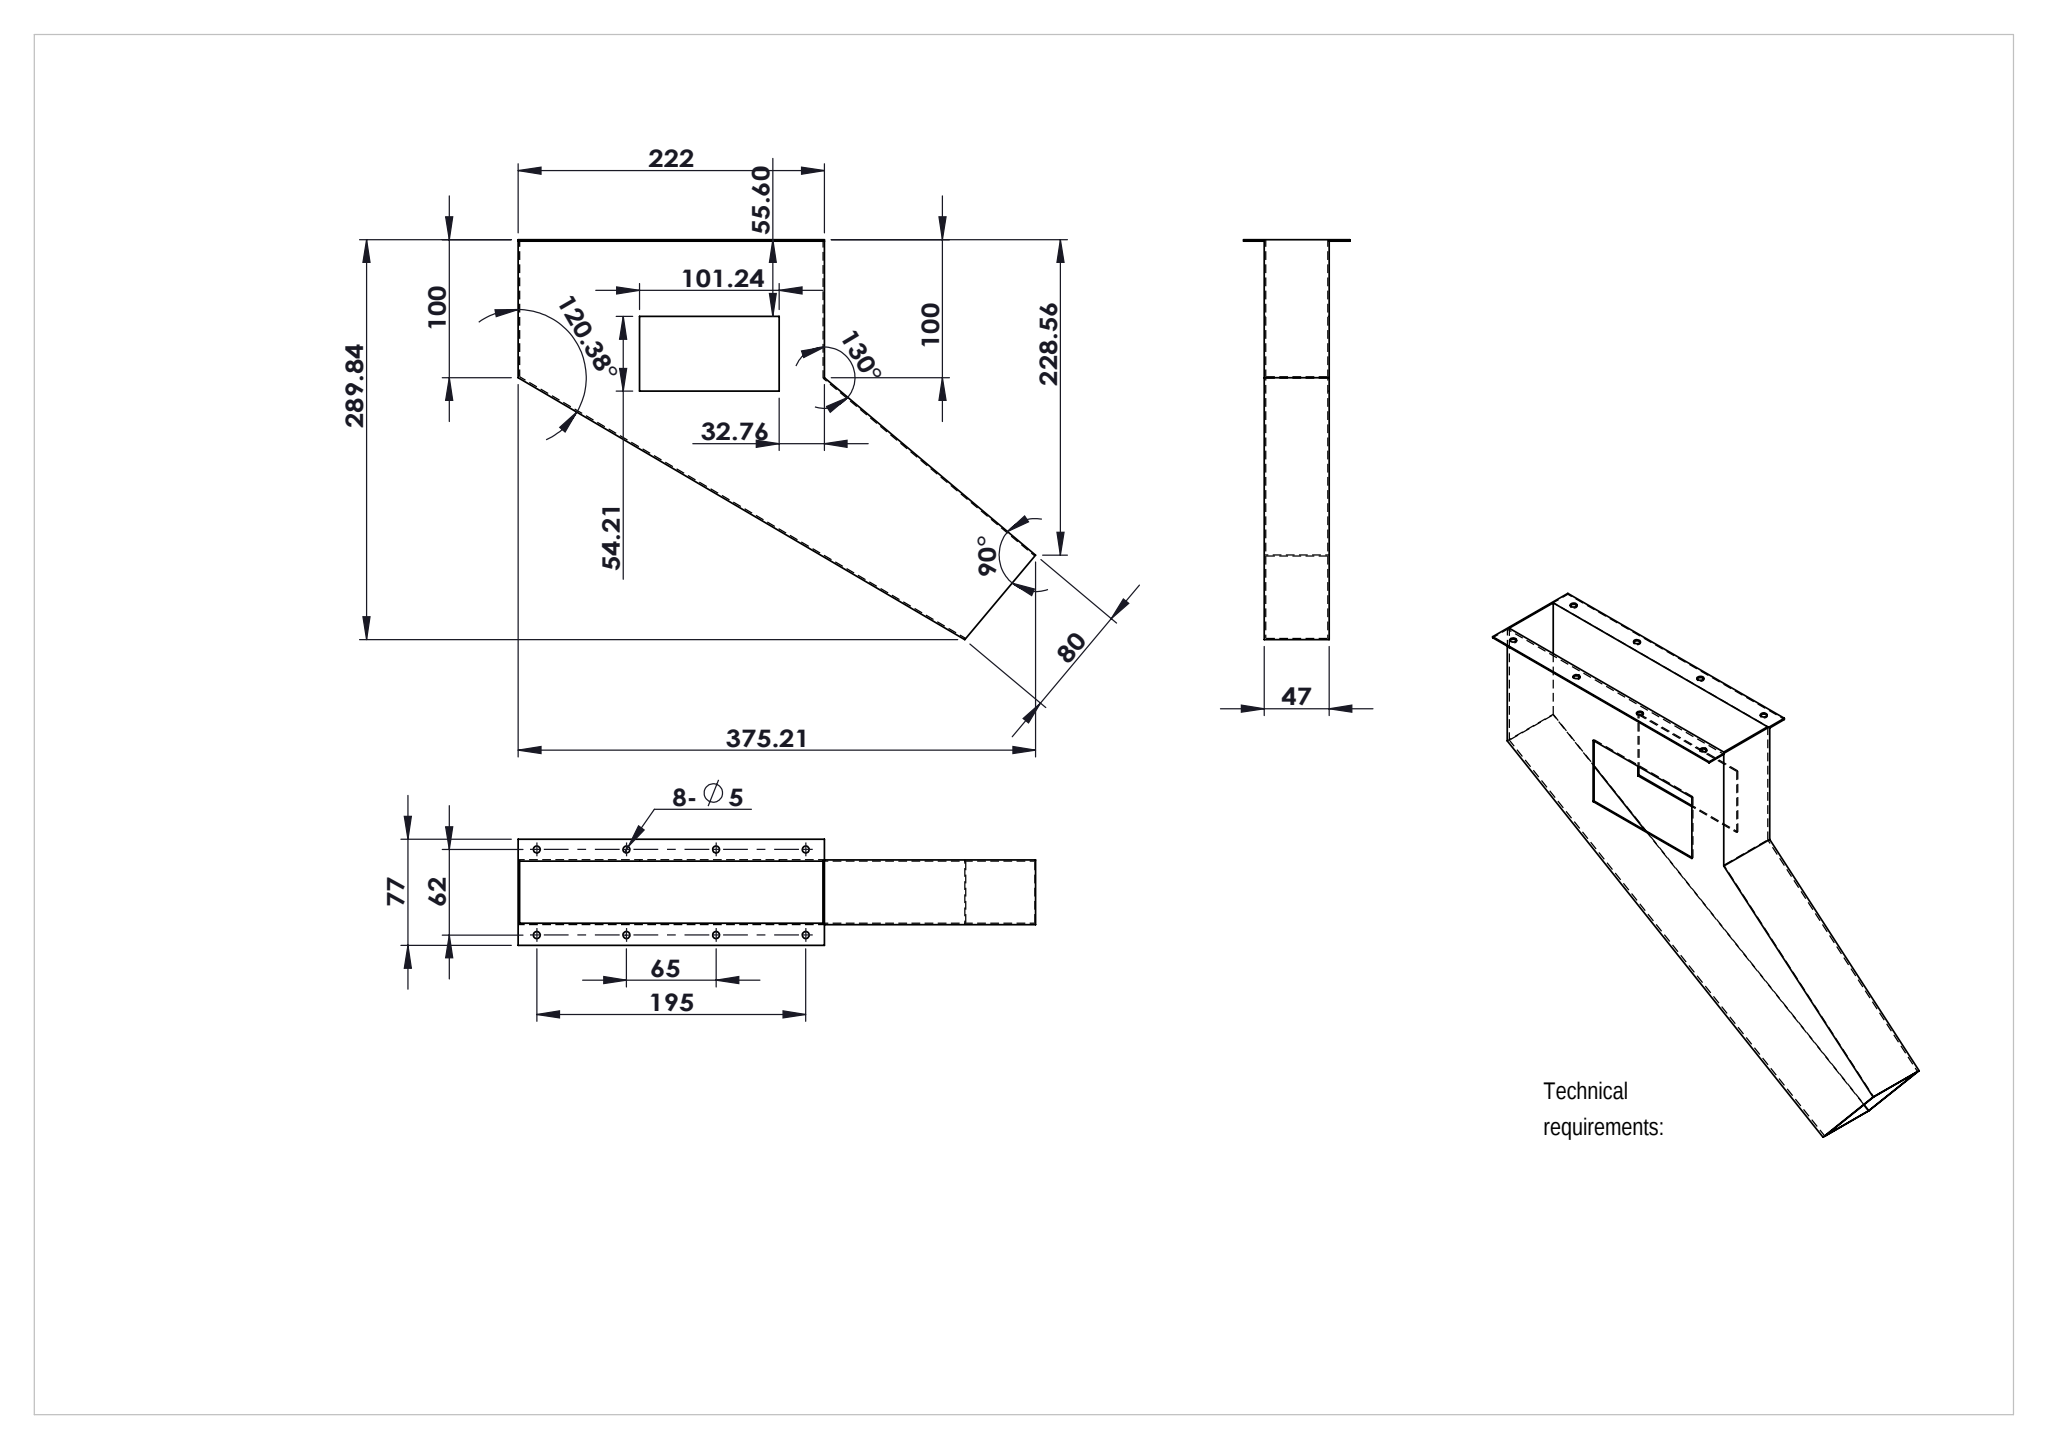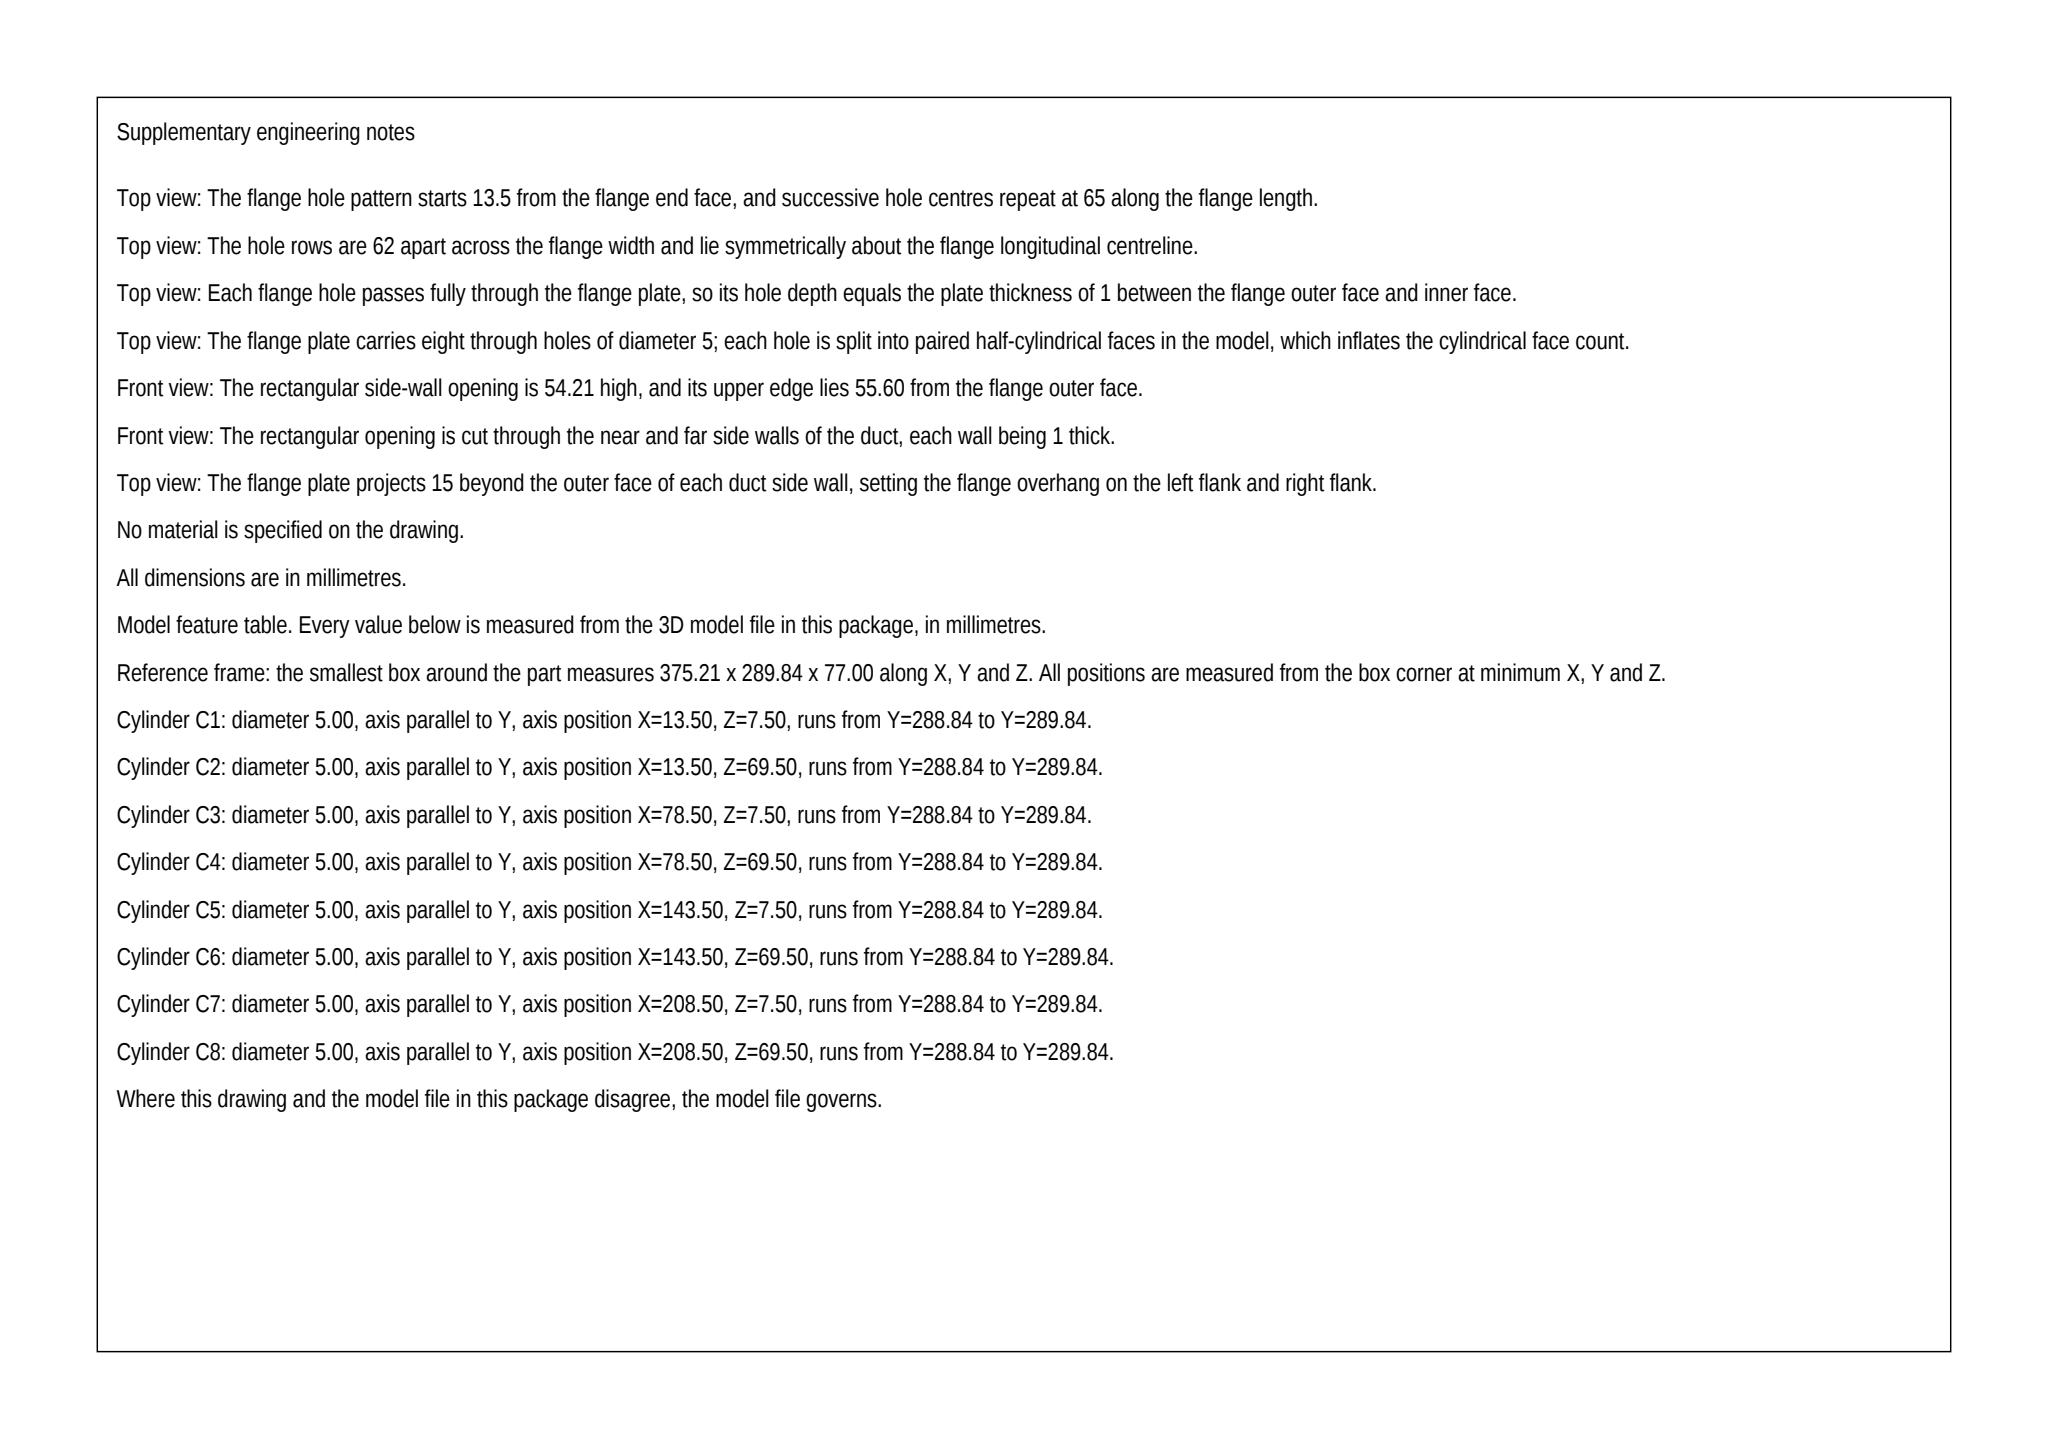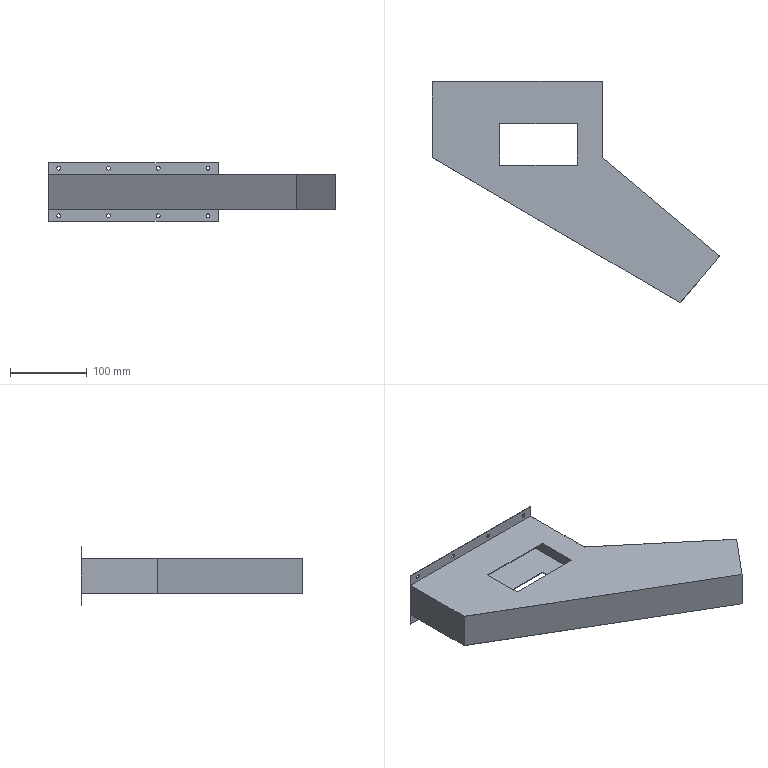Part | SolidWorks | mm | 1 solid | 42 faces | box 375.21 x 289.84 x 77 mm | volume 132960 mm3 | plane 26 | cylinder 16 | commonest cylinder face diameters 5 x16
Drawing notes:
8-Ø5: END HOLE CL 13.5 FROM FLANGE END, 65 PITCH | from the solid: Ø5 holes at x=13.5, 78.5, 143.5, 208.5 (65 spacing), z=7.5 & 69.5
SHEET THK 1 MM ALL DUCT WALLS & FLANGE | from the solid: Parallel face pairs offset 1 mm: z=15/16, z=61/62, x=0/1, x=221/222, y=288.8/289.8
ALL DIMS IN MM UNLESS OTHERWISE NOTED | from the solid: STEP model units mm; bbox 375.209 x 289.841 x 77.0
build123d program:
from build123d import *

# Parameters (mm, degrees)
BOSS_EXTRUDE1_DEPTH  = 23.5
SHELL1_T             = -1
SKETCH2_W            = 222
SKETCH2_H            = 1
BOSS_EXTRUDE2_DEPTH  = 15
SKETCH3_R            = 2.5
CUT_EXTRUDE1_DEPTH   = 367.327
LPATTERN1_COUNT      = 4
LPATTERN1_PITCH      = 65
SKETCH1_2_W          = 101.241
SKETCH1_2_H          = 54.213
CUT_EXTRUDE1_2_DEPTH = 220


with BuildPart() as part:
    # Sketch1 → Boss-Extrude1 (new, symmetric)
    with BuildSketch(Plane.XY):
        Polygon((0, 100), (0, 0), (153.209, -128.558), (101.786, -189.841), (-222, 0), (-222, 100), align=None)
    extrude(amount=BOSS_EXTRUDE1_DEPTH, both=True)

    # Shell1
    shell1_openings = [part.faces().sort_by_distance(p)[0] for p in [
        (127.497, -159.199, 0),
        (-111, 100, 0),
    ]]
    offset(amount=SHELL1_T, openings=shell1_openings, kind=Kind.INTERSECTION)

    # Sketch2 → Boss-Extrude2 (add)
    with BuildSketch(Plane.XY.offset(23.5)):
        with Locations((-111, 99.5)):
            Rectangle(SKETCH2_W, SKETCH2_H)
    boss_extrude2 = extrude(amount=BOSS_EXTRUDE2_DEPTH)

    # Mirror1: Boss-Extrude2 across plane
    add(boss_extrude2.mirror(Plane.XY))

    # Sketch3 → Cut-Extrude1 (cut, through all)
    with BuildSketch(Plane.XZ.offset(-99)):
        with Locations(Location((-208.5, 31, 0), (0, 0, 270))):
            Circle(SKETCH3_R)
        with Locations(Location((-208.5, -31, 0), (0, 0, 90))):
            Circle(SKETCH3_R)
    cut_extrude1 = extrude(amount=-CUT_EXTRUDE1_DEPTH, mode=Mode.SUBTRACT)

    # LPattern1: Cut-Extrude1 ×4
    with Locations(*[(i * LPATTERN1_PITCH, 0, 0) for i in range(1, LPATTERN1_COUNT)]):
        add(cut_extrude1, mode=Mode.SUBTRACT)

    # Sketch1_2 → Cut-Extrude1_2 (cut)
    with BuildSketch(Plane.XY.offset(23.5)):
        with Locations((-83.383, 17.293)):
            Rectangle(SKETCH1_2_W, SKETCH1_2_H)
    extrude(amount=-CUT_EXTRUDE1_2_DEPTH, mode=Mode.SUBTRACT)


solid = part.part